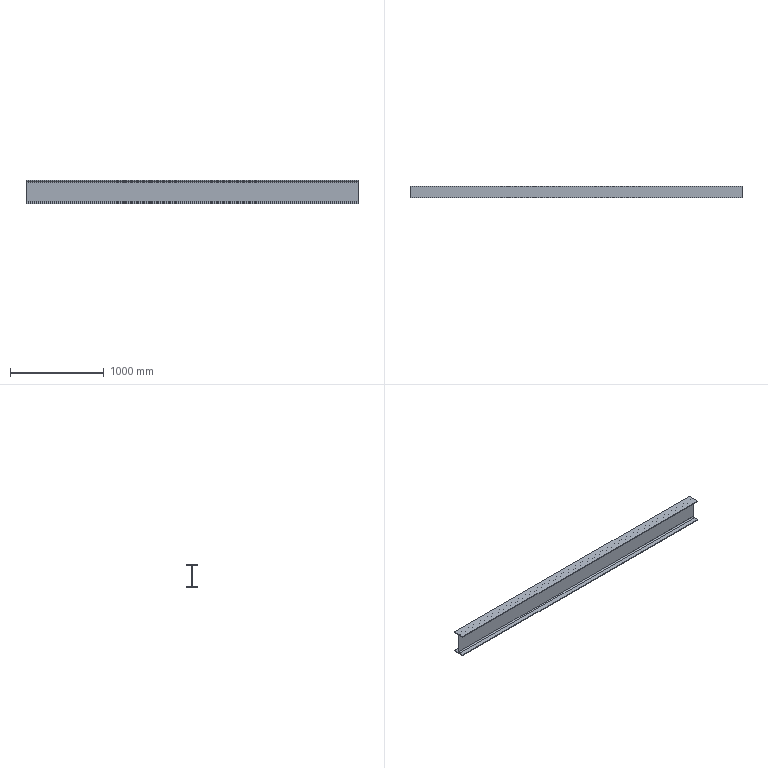Component | SolidWorks | H200X100-3600-13 | 1 solid | 18 faces | box 3550 x 125 x 250 mm | volume 12183851 mm3 | plane 14 | cylinder 4 | commonest cylinder face diameters 26 x4
build123d program:
from build123d import *

# Parameters (mm, degrees)
H_BEAM_HN200_100_1_DEPTH = 3550


with BuildPart() as part:
    # Sketch1 → H-beam HN200_100_1 (new body)
    with BuildSketch(Plane.YZ):
        with BuildLine():
            Line((-62.5, -125), (-62.5, -117))
            Line((-62.5, -117), (-15.75, -117))
            ThreePointArc((-15.75, -117), (-6.558, -113.192), (-2.75, -104))
            Line((-2.75, -104), (-2.75, 104))
            ThreePointArc((-2.75, 104), (-6.558, 113.192), (-15.75, 117))
            Line((-15.75, 117), (-62.5, 117))
            Line((-62.5, 117), (-62.5, 125))
            Line((-62.5, 125), (62.5, 125))
            Line((62.5, 125), (62.5, 117))
            Line((62.5, 117), (15.75, 117))
            ThreePointArc((15.75, 117), (6.558, 113.192), (2.75, 104))
            Line((2.75, 104), (2.75, -104))
            ThreePointArc((2.75, -104), (6.558, -113.192), (15.75, -117))
            Line((15.75, -117), (62.5, -117))
            Line((62.5, -117), (62.5, -125))
            Line((62.5, -125), (-62.5, -125))
        make_face()
    extrude(amount=H_BEAM_HN200_100_1_DEPTH)


solid = part.part

# Placed as in the assembly
solid = solid.moved(Location((-1730.074, -31202.346, 5154), (0, 0, 0)))
STEP:
#1=CARTESIAN_POINT('',(-68.113,-1230.899,197.992));
#2=VERTEX_POINT('',#1);
#3=CARTESIAN_POINT('',(-68.113,-1225.978,197.992));
#4=VERTEX_POINT('',#3);
#5=CARTESIAN_POINT('',(-68.113,-1225.978,197.992));
#6=DIRECTION('',(0.,1.,0.));
#7=VECTOR('',#6,39.37);
#8=LINE('',#5,#7);
#9=EDGE_CURVE('',#2,#4,#8,.T.);
#10=ORIENTED_EDGE('',*,*,#9,.T.);
#11=CARTESIAN_POINT('',(71.651,-1225.978,197.992));
#12=VERTEX_POINT('',#11);
#13=CARTESIAN_POINT('',(71.651,-1225.978,197.992));
#14=DIRECTION('',(-1.,0.,0.));
#15=VECTOR('',#14,39.37);
#16=LINE('',#13,#15);
#17=EDGE_CURVE('',#12,#4,#16,.T.);
#18=ORIENTED_EDGE('',*,*,#17,.F.);
#19=CARTESIAN_POINT('',(71.651,-1230.899,197.992));
#20=VERTEX_POINT('',#19);
#21=CARTESIAN_POINT('',(71.651,-1225.978,197.992));
#22=DIRECTION('',(0.,1.,0.));
#23=VECTOR('',#22,39.37);
#24=LINE('',#21,#23);
#25=EDGE_CURVE('',#20,#12,#24,.T.);
#26=ORIENTED_EDGE('',*,*,#25,.F.);
#27=CARTESIAN_POINT('',(71.651,-1230.899,197.992));
#28=DIRECTION('',(-1.,0.,0.));
#29=VECTOR('',#28,39.37);
#30=LINE('',#27,#29);
#31=EDGE_CURVE('',#20,#2,#30,.T.);
#32=ORIENTED_EDGE('',*,*,#31,.T.);
#33=EDGE_LOOP('',(#10,#18,#26,#32));
#34=FACE_OUTER_BOUND('',#33,.T.);
#35=CARTESIAN_POINT('',(71.651,-1225.978,197.992));
#36=DIRECTION('',(0.,0.,1.));
#37=DIRECTION('',(1.,0.,0.));
#38=AXIS2_PLACEMENT_3D('',#35,#36,#37);
#39=PLANE('',#38);
#40=ADVANCED_FACE('',(#34),#39,.F.);
#41=CARTESIAN_POINT('',(-68.113,-1225.978,198.307));
#42=VERTEX_POINT('',#41);
#43=CARTESIAN_POINT('',(-68.113,-1225.978,198.307));
#44=DIRECTION('',(0.,0.,1.));
#45=VECTOR('',#44,39.37);
#46=LINE('',#43,#45);
#47=EDGE_CURVE('',#4,#42,#46,.T.);
#48=ORIENTED_EDGE('',*,*,#47,.T.);
#49=CARTESIAN_POINT('',(71.651,-1225.978,198.307));
#50=VERTEX_POINT('',#49);
#51=CARTESIAN_POINT('',(71.651,-1225.978,198.307));
#52=DIRECTION('',(-1.,0.,0.));
#53=VECTOR('',#52,39.37);
#54=LINE('',#51,#53);
#55=EDGE_CURVE('',#50,#42,#54,.T.);
#56=ORIENTED_EDGE('',*,*,#55,.F.);
#57=CARTESIAN_POINT('',(71.651,-1225.978,198.307));
#58=DIRECTION('',(0.,0.,1.));
#59=VECTOR('',#58,39.37);
#60=LINE('',#57,#59);
#61=EDGE_CURVE('',#12,#50,#60,.T.);
#62=ORIENTED_EDGE('',*,*,#61,.F.);
#63=ORIENTED_EDGE('',*,*,#17,.T.);
#64=EDGE_LOOP('',(#48,#56,#62,#63));
#65=FACE_OUTER_BOUND('',#64,.T.);
#66=CARTESIAN_POINT('',(71.651,-1225.978,198.307));
#67=DIRECTION('',(0.,-1.,0.));
#68=DIRECTION('',(0.,0.,-1.));
#69=AXIS2_PLACEMENT_3D('',#66,#67,#68);
#70=PLANE('',#69);
#71=ADVANCED_FACE('',(#65),#70,.F.);
#72=CARTESIAN_POINT('',(-68.113,-1227.819,198.307));
#73=VERTEX_POINT('',#72);
#74=CARTESIAN_POINT('',(-68.113,-1225.978,198.307));
#75=DIRECTION('',(0.,-1.,0.));
#76=VECTOR('',#75,39.37);
#77=LINE('',#74,#76);
#78=EDGE_CURVE('',#42,#73,#77,.T.);
#79=ORIENTED_EDGE('',*,*,#78,.T.);
#80=CARTESIAN_POINT('',(71.651,-1227.819,198.307));
#81=VERTEX_POINT('',#80);
#82=CARTESIAN_POINT('',(71.651,-1227.819,198.307));
#83=DIRECTION('',(-1.,0.,0.));
#84=VECTOR('',#83,39.37);
#85=LINE('',#82,#84);
#86=EDGE_CURVE('',#81,#73,#85,.T.);
#87=ORIENTED_EDGE('',*,*,#86,.F.);
#88=CARTESIAN_POINT('',(71.651,-1225.978,198.307));
#89=DIRECTION('',(0.,-1.,0.));
#90=VECTOR('',#89,39.37);
#91=LINE('',#88,#90);
#92=EDGE_CURVE('',#50,#81,#91,.T.);
#93=ORIENTED_EDGE('',*,*,#92,.F.);
#94=ORIENTED_EDGE('',*,*,#55,.T.);
#95=EDGE_LOOP('',(#79,#87,#93,#94));
#96=FACE_OUTER_BOUND('',#95,.T.);
#97=CARTESIAN_POINT('',(71.651,-1225.978,198.307));
#98=DIRECTION('',(0.,0.,-1.));
#99=DIRECTION('',(-1.,0.,0.));
#100=AXIS2_PLACEMENT_3D('',#97,#98,#99);
#101=PLANE('',#100);
#102=ADVANCED_FACE('',(#96),#101,.F.);
#103=CARTESIAN_POINT('',(-68.113,-1228.331,198.819));
#104=VERTEX_POINT('',#103);
#105=CARTESIAN_POINT('',(-68.113,-1227.819,198.819));
#106=DIRECTION('',(-1.,0.,0.));
#107=DIRECTION('',(0.,0.,1.));
#108=AXIS2_PLACEMENT_3D('',#105,#106,#107);
#109=CIRCLE('',#108,0.5118);
#110=EDGE_CURVE('',#73,#104,#109,.T.);
#111=ORIENTED_EDGE('',*,*,#110,.T.);
#112=CARTESIAN_POINT('',(71.651,-1228.331,198.819));
#113=VERTEX_POINT('',#112);
#114=CARTESIAN_POINT('',(71.651,-1228.331,198.819));
#115=DIRECTION('',(-1.,0.,0.));
#116=VECTOR('',#115,39.37);
#117=LINE('',#114,#116);
#118=EDGE_CURVE('',#113,#104,#117,.T.);
#119=ORIENTED_EDGE('',*,*,#118,.F.);
#120=CARTESIAN_POINT('',(71.651,-1227.819,198.819));
#121=DIRECTION('',(-1.,0.,0.));
#122=DIRECTION('',(0.,0.,1.));
#123=AXIS2_PLACEMENT_3D('',#120,#121,#122);
#124=CIRCLE('',#123,0.5118);
#125=EDGE_CURVE('',#81,#113,#124,.T.);
#126=ORIENTED_EDGE('',*,*,#125,.F.);
#127=ORIENTED_EDGE('',*,*,#86,.T.);
#128=EDGE_LOOP('',(#111,#119,#126,#127));
#129=FACE_OUTER_BOUND('',#128,.T.);
#130=CARTESIAN_POINT('',(71.651,-1227.819,198.819));
#131=DIRECTION('',(-1.,0.,0.));
#132=DIRECTION('',(0.,0.,1.));
#133=AXIS2_PLACEMENT_3D('',#130,#131,#132);
#134=CYLINDRICAL_SURFACE('',#133,0.5118);
#135=ADVANCED_FACE('',(#129),#134,.F.);
#136=CARTESIAN_POINT('',(-68.113,-1228.331,207.008));
#137=VERTEX_POINT('',#136);
#138=CARTESIAN_POINT('',(-68.113,-1228.331,207.008));
#139=DIRECTION('',(0.,-0.,1.));
#140=VECTOR('',#139,39.37);
#141=LINE('',#138,#140);
#142=EDGE_CURVE('',#104,#137,#141,.T.);
#143=ORIENTED_EDGE('',*,*,#142,.T.);
#144=CARTESIAN_POINT('',(71.651,-1228.331,207.008));
#145=VERTEX_POINT('',#144);
#146=CARTESIAN_POINT('',(71.651,-1228.331,207.008));
#147=DIRECTION('',(-1.,0.,0.));
#148=VECTOR('',#147,39.37);
#149=LINE('',#146,#148);
#150=EDGE_CURVE('',#145,#137,#149,.T.);
#151=ORIENTED_EDGE('',*,*,#150,.F.);
#152=CARTESIAN_POINT('',(71.651,-1228.331,207.008));
#153=DIRECTION('',(0.,-0.,1.));
#154=VECTOR('',#153,39.37);
#155=LINE('',#152,#154);
#156=EDGE_CURVE('',#113,#145,#155,.T.);
#157=ORIENTED_EDGE('',*,*,#156,.F.);
#158=ORIENTED_EDGE('',*,*,#118,.T.);
#159=EDGE_LOOP('',(#143,#151,#157,#158));
#160=FACE_OUTER_BOUND('',#159,.T.);
#161=CARTESIAN_POINT('',(71.651,-1228.331,207.008));
#162=DIRECTION('',(0.,-1.,-0.));
#163=DIRECTION('',(0.,0.,-1.));
#164=AXIS2_PLACEMENT_3D('',#161,#162,#163);
#165=PLANE('',#164);
#166=ADVANCED_FACE('',(#160),#165,.F.);
#167=CARTESIAN_POINT('',(-68.113,-1227.819,207.52));
#168=VERTEX_POINT('',#167);
#169=CARTESIAN_POINT('',(-68.113,-1227.819,207.008));
#170=DIRECTION('',(-1.,0.,0.));
#171=DIRECTION('',(0.,0.,1.));
#172=AXIS2_PLACEMENT_3D('',#169,#170,#171);
#173=CIRCLE('',#172,0.5118);
#174=EDGE_CURVE('',#137,#168,#173,.T.);
#175=ORIENTED_EDGE('',*,*,#174,.T.);
#176=CARTESIAN_POINT('',(71.651,-1227.819,207.52));
#177=VERTEX_POINT('',#176);
#178=CARTESIAN_POINT('',(71.651,-1227.819,207.52));
#179=DIRECTION('',(-1.,0.,0.));
#180=VECTOR('',#179,39.37);
#181=LINE('',#178,#180);
#182=EDGE_CURVE('',#177,#168,#181,.T.);
#183=ORIENTED_EDGE('',*,*,#182,.F.);
#184=CARTESIAN_POINT('',(71.651,-1227.819,207.008));
#185=DIRECTION('',(-1.,0.,0.));
#186=DIRECTION('',(0.,0.,1.));
#187=AXIS2_PLACEMENT_3D('',#184,#185,#186);
#188=CIRCLE('',#187,0.5118);
#189=EDGE_CURVE('',#145,#177,#188,.T.);
#190=ORIENTED_EDGE('',*,*,#189,.F.);
#191=ORIENTED_EDGE('',*,*,#150,.T.);
#192=EDGE_LOOP('',(#175,#183,#190,#191));
#193=FACE_OUTER_BOUND('',#192,.T.);
#194=CARTESIAN_POINT('',(71.651,-1227.819,207.008));
#195=DIRECTION('',(-1.,0.,0.));
#196=DIRECTION('',(0.,0.,1.));
#197=AXIS2_PLACEMENT_3D('',#194,#195,#196);
#198=CYLINDRICAL_SURFACE('',#197,0.5118);
#199=ADVANCED_FACE('',(#193),#198,.F.);
#200=CARTESIAN_POINT('',(-68.113,-1225.978,207.52));
#201=VERTEX_POINT('',#200);
#202=CARTESIAN_POINT('',(-68.113,-1227.819,207.52));
#203=DIRECTION('',(0.,1.,0.));
#204=VECTOR('',#203,39.37);
#205=LINE('',#202,#204);
#206=EDGE_CURVE('',#168,#201,#205,.T.);
#207=ORIENTED_EDGE('',*,*,#206,.T.);
#208=CARTESIAN_POINT('',(71.651,-1225.978,207.52));
#209=VERTEX_POINT('',#208);
#210=CARTESIAN_POINT('',(71.651,-1225.978,207.52));
#211=DIRECTION('',(-1.,0.,0.));
#212=VECTOR('',#211,39.37);
#213=LINE('',#210,#212);
#214=EDGE_CURVE('',#209,#201,#213,.T.);
#215=ORIENTED_EDGE('',*,*,#214,.F.);
#216=CARTESIAN_POINT('',(71.651,-1227.819,207.52));
#217=DIRECTION('',(0.,1.,0.));
#218=VECTOR('',#217,39.37);
#219=LINE('',#216,#218);
#220=EDGE_CURVE('',#177,#209,#219,.T.);
#221=ORIENTED_EDGE('',*,*,#220,.F.);
#222=ORIENTED_EDGE('',*,*,#182,.T.);
#223=EDGE_LOOP('',(#207,#215,#221,#222));
#224=FACE_OUTER_BOUND('',#223,.T.);
#225=CARTESIAN_POINT('',(71.651,-1227.819,207.52));
#226=DIRECTION('',(0.,0.,1.));
#227=DIRECTION('',(1.,0.,0.));
#228=AXIS2_PLACEMENT_3D('',#225,#226,#227);
#229=PLANE('',#228);
#230=ADVANCED_FACE('',(#224),#229,.F.);
#231=CARTESIAN_POINT('',(-68.113,-1225.978,207.835));
#232=VERTEX_POINT('',#231);
#233=CARTESIAN_POINT('',(-68.113,-1225.978,207.835));
#234=DIRECTION('',(0.,0.,1.));
#235=VECTOR('',#234,39.37);
#236=LINE('',#233,#235);
#237=EDGE_CURVE('',#201,#232,#236,.T.);
#238=ORIENTED_EDGE('',*,*,#237,.T.);
#239=CARTESIAN_POINT('',(71.651,-1225.978,207.835));
#240=VERTEX_POINT('',#239);
#241=CARTESIAN_POINT('',(71.651,-1225.978,207.835));
#242=DIRECTION('',(-1.,0.,0.));
#243=VECTOR('',#242,39.37);
#244=LINE('',#241,#243);
#245=EDGE_CURVE('',#240,#232,#244,.T.);
#246=ORIENTED_EDGE('',*,*,#245,.F.);
#247=CARTESIAN_POINT('',(71.651,-1225.978,207.835));
#248=DIRECTION('',(0.,0.,1.));
#249=VECTOR('',#248,39.37);
#250=LINE('',#247,#249);
#251=EDGE_CURVE('',#209,#240,#250,.T.);
#252=ORIENTED_EDGE('',*,*,#251,.F.);
#253=ORIENTED_EDGE('',*,*,#214,.T.);
#254=EDGE_LOOP('',(#238,#246,#252,#253));
#255=FACE_OUTER_BOUND('',#254,.T.);
#256=CARTESIAN_POINT('',(71.651,-1225.978,207.835));
#257=DIRECTION('',(0.,-1.,0.));
#258=DIRECTION('',(0.,0.,-1.));
#259=AXIS2_PLACEMENT_3D('',#256,#257,#258);
#260=PLANE('',#259);
#261=ADVANCED_FACE('',(#255),#260,.F.);
#262=CARTESIAN_POINT('',(-68.113,-1230.899,207.835));
#263=VERTEX_POINT('',#262);
#264=CARTESIAN_POINT('',(-68.113,-1230.899,207.835));
#265=DIRECTION('',(0.,-1.,0.));
#266=VECTOR('',#265,39.37);
#267=LINE('',#264,#266);
#268=EDGE_CURVE('',#232,#263,#267,.T.);
#269=ORIENTED_EDGE('',*,*,#268,.T.);
#270=CARTESIAN_POINT('',(71.651,-1230.899,207.835));
#271=VERTEX_POINT('',#270);
#272=CARTESIAN_POINT('',(71.651,-1230.899,207.835));
#273=DIRECTION('',(-1.,0.,0.));
#274=VECTOR('',#273,39.37);
#275=LINE('',#272,#274);
#276=EDGE_CURVE('',#271,#263,#275,.T.);
#277=ORIENTED_EDGE('',*,*,#276,.F.);
#278=CARTESIAN_POINT('',(71.651,-1230.899,207.835));
#279=DIRECTION('',(0.,-1.,0.));
#280=VECTOR('',#279,39.37);
#281=LINE('',#278,#280);
#282=EDGE_CURVE('',#240,#271,#281,.T.);
#283=ORIENTED_EDGE('',*,*,#282,.F.);
#284=ORIENTED_EDGE('',*,*,#245,.T.);
#285=EDGE_LOOP('',(#269,#277,#283,#284));
#286=FACE_OUTER_BOUND('',#285,.T.);
#287=CARTESIAN_POINT('',(71.651,-1230.899,207.835));
#288=DIRECTION('',(0.,0.,-1.));
#289=DIRECTION('',(-1.,0.,0.));
#290=AXIS2_PLACEMENT_3D('',#287,#288,#289);
#291=PLANE('',#290);
#292=ADVANCED_FACE('',(#286),#291,.F.);
#293=CARTESIAN_POINT('',(-68.113,-1230.899,207.52));
#294=VERTEX_POINT('',#293);
#295=CARTESIAN_POINT('',(-68.113,-1230.899,207.52));
#296=DIRECTION('',(0.,0.,-1.));
#297=VECTOR('',#296,39.37);
#298=LINE('',#295,#297);
#299=EDGE_CURVE('',#263,#294,#298,.T.);
#300=ORIENTED_EDGE('',*,*,#299,.T.);
#301=CARTESIAN_POINT('',(71.651,-1230.899,207.52));
#302=VERTEX_POINT('',#301);
#303=CARTESIAN_POINT('',(71.651,-1230.899,207.52));
#304=DIRECTION('',(-1.,0.,0.));
#305=VECTOR('',#304,39.37);
#306=LINE('',#303,#305);
#307=EDGE_CURVE('',#302,#294,#306,.T.);
#308=ORIENTED_EDGE('',*,*,#307,.F.);
#309=CARTESIAN_POINT('',(71.651,-1230.899,207.52));
#310=DIRECTION('',(0.,0.,-1.));
#311=VECTOR('',#310,39.37);
#312=LINE('',#309,#311);
#313=EDGE_CURVE('',#271,#302,#312,.T.);
#314=ORIENTED_EDGE('',*,*,#313,.F.);
#315=ORIENTED_EDGE('',*,*,#276,.T.);
#316=EDGE_LOOP('',(#300,#308,#314,#315));
#317=FACE_OUTER_BOUND('',#316,.T.);
#318=CARTESIAN_POINT('',(71.651,-1230.899,207.52));
#319=DIRECTION('',(0.,1.,0.));
#320=DIRECTION('',(0.,0.,1.));
#321=AXIS2_PLACEMENT_3D('',#318,#319,#320);
#322=PLANE('',#321);
#323=ADVANCED_FACE('',(#317),#322,.F.);
#324=CARTESIAN_POINT('',(-68.113,-1229.059,207.52));
#325=VERTEX_POINT('',#324);
#326=CARTESIAN_POINT('',(-68.113,-1230.899,207.52));
#327=DIRECTION('',(0.,1.,0.));
#328=VECTOR('',#327,39.37);
#329=LINE('',#326,#328);
#330=EDGE_CURVE('',#294,#325,#329,.T.);
#331=ORIENTED_EDGE('',*,*,#330,.T.);
#332=CARTESIAN_POINT('',(71.651,-1229.059,207.52));
#333=VERTEX_POINT('',#332);
#334=CARTESIAN_POINT('',(71.651,-1229.059,207.52));
#335=DIRECTION('',(-1.,0.,0.));
#336=VECTOR('',#335,39.37);
#337=LINE('',#334,#336);
#338=EDGE_CURVE('',#333,#325,#337,.T.);
#339=ORIENTED_EDGE('',*,*,#338,.F.);
#340=CARTESIAN_POINT('',(71.651,-1230.899,207.52));
#341=DIRECTION('',(0.,1.,0.));
#342=VECTOR('',#341,39.37);
#343=LINE('',#340,#342);
#344=EDGE_CURVE('',#302,#333,#343,.T.);
#345=ORIENTED_EDGE('',*,*,#344,.F.);
#346=ORIENTED_EDGE('',*,*,#307,.T.);
#347=EDGE_LOOP('',(#331,#339,#345,#346));
#348=FACE_OUTER_BOUND('',#347,.T.);
#349=CARTESIAN_POINT('',(71.651,-1230.899,207.52));
#350=DIRECTION('',(0.,0.,1.));
#351=DIRECTION('',(1.,0.,0.));
#352=AXIS2_PLACEMENT_3D('',#349,#350,#351);
#353=PLANE('',#352);
#354=ADVANCED_FACE('',(#348),#353,.F.);
#355=CARTESIAN_POINT('',(-68.113,-1228.547,207.008));
#356=VERTEX_POINT('',#355);
#357=CARTESIAN_POINT('',(-68.113,-1229.059,207.008));
#358=DIRECTION('',(-1.,0.,0.));
#359=DIRECTION('',(0.,0.,-1.));
#360=AXIS2_PLACEMENT_3D('',#357,#358,#359);
#361=CIRCLE('',#360,0.5118);
#362=EDGE_CURVE('',#325,#356,#361,.T.);
#363=ORIENTED_EDGE('',*,*,#362,.T.);
#364=CARTESIAN_POINT('',(71.651,-1228.547,207.008));
#365=VERTEX_POINT('',#364);
#366=CARTESIAN_POINT('',(71.651,-1228.547,207.008));
#367=DIRECTION('',(-1.,0.,0.));
#368=VECTOR('',#367,39.37);
#369=LINE('',#366,#368);
#370=EDGE_CURVE('',#365,#356,#369,.T.);
#371=ORIENTED_EDGE('',*,*,#370,.F.);
#372=CARTESIAN_POINT('',(71.651,-1229.059,207.008));
#373=DIRECTION('',(-1.,0.,0.));
#374=DIRECTION('',(0.,0.,-1.));
#375=AXIS2_PLACEMENT_3D('',#372,#373,#374);
#376=CIRCLE('',#375,0.5118);
#377=EDGE_CURVE('',#333,#365,#376,.T.);
#378=ORIENTED_EDGE('',*,*,#377,.F.);
#379=ORIENTED_EDGE('',*,*,#338,.T.);
#380=EDGE_LOOP('',(#363,#371,#378,#379));
#381=FACE_OUTER_BOUND('',#380,.T.);
#382=CARTESIAN_POINT('',(71.651,-1229.059,207.008));
#383=DIRECTION('',(-1.,0.,0.));
#384=DIRECTION('',(0.,0.,1.));
#385=AXIS2_PLACEMENT_3D('',#382,#383,#384);
#386=CYLINDRICAL_SURFACE('',#385,0.5118);
#387=ADVANCED_FACE('',(#381),#386,.F.);
#388=CARTESIAN_POINT('',(-68.113,-1228.547,198.819));
#389=VERTEX_POINT('',#388);
#390=CARTESIAN_POINT('',(-68.113,-1228.547,198.819));
#391=DIRECTION('',(0.,0.,-1.));
#392=VECTOR('',#391,39.37);
#393=LINE('',#390,#392);
#394=EDGE_CURVE('',#356,#389,#393,.T.);
#395=ORIENTED_EDGE('',*,*,#394,.T.);
#396=CARTESIAN_POINT('',(71.651,-1228.547,198.819));
#397=VERTEX_POINT('',#396);
#398=CARTESIAN_POINT('',(71.651,-1228.547,198.819));
#399=DIRECTION('',(-1.,0.,0.));
#400=VECTOR('',#399,39.37);
#401=LINE('',#398,#400);
#402=EDGE_CURVE('',#397,#389,#401,.T.);
#403=ORIENTED_EDGE('',*,*,#402,.F.);
#404=CARTESIAN_POINT('',(71.651,-1228.547,198.819));
#405=DIRECTION('',(0.,0.,-1.));
#406=VECTOR('',#405,39.37);
#407=LINE('',#404,#406);
#408=EDGE_CURVE('',#365,#397,#407,.T.);
#409=ORIENTED_EDGE('',*,*,#408,.F.);
#410=ORIENTED_EDGE('',*,*,#370,.T.);
#411=EDGE_LOOP('',(#395,#403,#409,#410));
#412=FACE_OUTER_BOUND('',#411,.T.);
#413=CARTESIAN_POINT('',(71.651,-1228.547,198.819));
#414=DIRECTION('',(0.,1.,0.));
#415=DIRECTION('',(0.,-0.,1.));
#416=AXIS2_PLACEMENT_3D('',#413,#414,#415);
#417=PLANE('',#416);
#418=ADVANCED_FACE('',(#412),#417,.F.);
#419=CARTESIAN_POINT('',(-68.113,-1229.059,198.307));
#420=VERTEX_POINT('',#419);
#421=CARTESIAN_POINT('',(-68.113,-1229.059,198.819));
#422=DIRECTION('',(-1.,0.,0.));
#423=DIRECTION('',(0.,0.,-1.));
#424=AXIS2_PLACEMENT_3D('',#421,#422,#423);
#425=CIRCLE('',#424,0.5118);
#426=EDGE_CURVE('',#389,#420,#425,.T.);
#427=ORIENTED_EDGE('',*,*,#426,.T.);
#428=CARTESIAN_POINT('',(71.651,-1229.059,198.307));
#429=VERTEX_POINT('',#428);
#430=CARTESIAN_POINT('',(71.651,-1229.059,198.307));
#431=DIRECTION('',(-1.,0.,0.));
#432=VECTOR('',#431,39.37);
#433=LINE('',#430,#432);
#434=EDGE_CURVE('',#429,#420,#433,.T.);
#435=ORIENTED_EDGE('',*,*,#434,.F.);
#436=CARTESIAN_POINT('',(71.651,-1229.059,198.819));
#437=DIRECTION('',(-1.,0.,0.));
#438=DIRECTION('',(0.,0.,-1.));
#439=AXIS2_PLACEMENT_3D('',#436,#437,#438);
#440=CIRCLE('',#439,0.5118);
#441=EDGE_CURVE('',#397,#429,#440,.T.);
#442=ORIENTED_EDGE('',*,*,#441,.F.);
#443=ORIENTED_EDGE('',*,*,#402,.T.);
#444=EDGE_LOOP('',(#427,#435,#442,#443));
#445=FACE_OUTER_BOUND('',#444,.T.);
#446=CARTESIAN_POINT('',(71.651,-1229.059,198.819));
#447=DIRECTION('',(-1.,0.,0.));
#448=DIRECTION('',(0.,0.,1.));
#449=AXIS2_PLACEMENT_3D('',#446,#447,#448);
#450=CYLINDRICAL_SURFACE('',#449,0.5118);
#451=ADVANCED_FACE('',(#445),#450,.F.);
#452=CARTESIAN_POINT('',(-68.113,-1230.899,198.307));
#453=VERTEX_POINT('',#452);
#454=CARTESIAN_POINT('',(-68.113,-1229.059,198.307));
#455=DIRECTION('',(0.,-1.,0.));
#456=VECTOR('',#455,39.37);
#457=LINE('',#454,#456);
#458=EDGE_CURVE('',#420,#453,#457,.T.);
#459=ORIENTED_EDGE('',*,*,#458,.T.);
#460=CARTESIAN_POINT('',(71.651,-1230.899,198.307));
#461=VERTEX_POINT('',#460);
#462=CARTESIAN_POINT('',(71.651,-1230.899,198.307));
#463=DIRECTION('',(-1.,0.,0.));
#464=VECTOR('',#463,39.37);
#465=LINE('',#462,#464);
#466=EDGE_CURVE('',#461,#453,#465,.T.);
#467=ORIENTED_EDGE('',*,*,#466,.F.);
#468=CARTESIAN_POINT('',(71.651,-1229.059,198.307));
#469=DIRECTION('',(0.,-1.,0.));
#470=VECTOR('',#469,39.37);
#471=LINE('',#468,#470);
#472=EDGE_CURVE('',#429,#461,#471,.T.);
#473=ORIENTED_EDGE('',*,*,#472,.F.);
#474=ORIENTED_EDGE('',*,*,#434,.T.);
#475=EDGE_LOOP('',(#459,#467,#473,#474));
#476=FACE_OUTER_BOUND('',#475,.T.);
#477=CARTESIAN_POINT('',(71.651,-1229.059,198.307));
#478=DIRECTION('',(0.,0.,-1.));
#479=DIRECTION('',(-1.,0.,0.));
#480=AXIS2_PLACEMENT_3D('',#477,#478,#479);
#481=PLANE('',#480);
#482=ADVANCED_FACE('',(#476),#481,.F.);
#483=CARTESIAN_POINT('',(-68.113,-1230.899,197.992));
#484=DIRECTION('',(0.,0.,-1.));
#485=VECTOR('',#484,39.37);
#486=LINE('',#483,#485);
#487=EDGE_CURVE('',#453,#2,#486,.T.);
#488=ORIENTED_EDGE('',*,*,#487,.T.);
#489=ORIENTED_EDGE('',*,*,#31,.F.);
#490=CARTESIAN_POINT('',(71.651,-1230.899,197.992));
#491=DIRECTION('',(0.,0.,-1.));
#492=VECTOR('',#491,39.37);
#493=LINE('',#490,#492);
#494=EDGE_CURVE('',#461,#20,#493,.T.);
#495=ORIENTED_EDGE('',*,*,#494,.F.);
#496=ORIENTED_EDGE('',*,*,#466,.T.);
#497=EDGE_LOOP('',(#488,#489,#495,#496));
#498=FACE_OUTER_BOUND('',#497,.T.);
#499=CARTESIAN_POINT('',(71.651,-1230.899,197.992));
#500=DIRECTION('',(0.,1.,0.));
#501=DIRECTION('',(0.,0.,1.));
#502=AXIS2_PLACEMENT_3D('',#499,#500,#501);
#503=PLANE('',#502);
#504=ADVANCED_FACE('',(#498),#503,.F.);
#505=ORIENTED_EDGE('',*,*,#25,.T.);
#506=ORIENTED_EDGE('',*,*,#61,.T.);
#507=ORIENTED_EDGE('',*,*,#92,.T.);
#508=ORIENTED_EDGE('',*,*,#125,.T.);
#509=ORIENTED_EDGE('',*,*,#156,.T.);
#510=ORIENTED_EDGE('',*,*,#189,.T.);
#511=ORIENTED_EDGE('',*,*,#220,.T.);
#512=ORIENTED_EDGE('',*,*,#251,.T.);
#513=ORIENTED_EDGE('',*,*,#282,.T.);
#514=ORIENTED_EDGE('',*,*,#313,.T.);
#515=ORIENTED_EDGE('',*,*,#344,.T.);
#516=ORIENTED_EDGE('',*,*,#377,.T.);
#517=ORIENTED_EDGE('',*,*,#408,.T.);
#518=ORIENTED_EDGE('',*,*,#441,.T.);
#519=ORIENTED_EDGE('',*,*,#472,.T.);
#520=ORIENTED_EDGE('',*,*,#494,.T.);
#521=EDGE_LOOP('',(#505,#506,#507,#508,#509,#510,#511,#512,#513,#514,#515,#516,#517,#518,#519,#520));
#522=FACE_OUTER_BOUND('',#521,.T.);
#523=CARTESIAN_POINT('',(71.651,-1229.059,198.819));
#524=DIRECTION('',(1.,0.,0.));
#525=DIRECTION('',(0.,0.,-1.));
#526=AXIS2_PLACEMENT_3D('',#523,#524,#525);
#527=PLANE('',#526);
#528=ADVANCED_FACE('',(#522),#527,.T.);
#529=ORIENTED_EDGE('',*,*,#9,.F.);
#530=ORIENTED_EDGE('',*,*,#487,.F.);
#531=ORIENTED_EDGE('',*,*,#458,.F.);
#532=ORIENTED_EDGE('',*,*,#426,.F.);
#533=ORIENTED_EDGE('',*,*,#394,.F.);
#534=ORIENTED_EDGE('',*,*,#362,.F.);
#535=ORIENTED_EDGE('',*,*,#330,.F.);
#536=ORIENTED_EDGE('',*,*,#299,.F.);
#537=ORIENTED_EDGE('',*,*,#268,.F.);
#538=ORIENTED_EDGE('',*,*,#237,.F.);
#539=ORIENTED_EDGE('',*,*,#206,.F.);
#540=ORIENTED_EDGE('',*,*,#174,.F.);
#541=ORIENTED_EDGE('',*,*,#142,.F.);
#542=ORIENTED_EDGE('',*,*,#110,.F.);
#543=ORIENTED_EDGE('',*,*,#78,.F.);
#544=ORIENTED_EDGE('',*,*,#47,.F.);
#545=EDGE_LOOP('',(#529,#530,#531,#532,#533,#534,#535,#536,#537,#538,#539,#540,#541,#542,#543,#544));
#546=FACE_OUTER_BOUND('',#545,.T.);
#547=CARTESIAN_POINT('',(-68.113,-1229.059,198.819));
#548=DIRECTION('',(1.,0.,0.));
#549=DIRECTION('',(0.,0.,-1.));
#550=AXIS2_PLACEMENT_3D('',#547,#548,#549);
#551=PLANE('',#550);
#552=ADVANCED_FACE('',(#546),#551,.F.);
#553=CLOSED_SHELL('',(#40,#71,#102,#135,#166,#199,#230,#261,#292,#323,#354,#387,#418,#451,#482,#504,#528,#552));
#554=MANIFOLD_SOLID_BREP('',#553);
#555=CARTESIAN_POINT('',(0.,0.,0.));
#556=DIRECTION('',(0.,0.,1.));
#557=DIRECTION('',(1.,0.,0.));
#558=AXIS2_PLACEMENT_3D('',#555,#556,#557);
#559=(LENGTH_UNIT()NAMED_UNIT(*)SI_UNIT($,.METRE.));
#560=LENGTH_MEASURE_WITH_UNIT(LENGTH_MEASURE(0.0254),#559);
#561=DIMENSIONAL_EXPONENTS(1.,0.,0.,0.,0.,0.,0.);
#562=(CONVERSION_BASED_UNIT('',#560)LENGTH_UNIT()NAMED_UNIT(#561));
#563=UNCERTAINTY_MEASURE_WITH_UNIT(LENGTH_MEASURE(0.00001),#562,'','');
#564=(NAMED_UNIT(*)PLANE_ANGLE_UNIT()SI_UNIT($,.RADIAN.));
#565=(NAMED_UNIT(*)SI_UNIT($,.STERADIAN.)SOLID_ANGLE_UNIT());
#566=(GEOMETRIC_REPRESENTATION_CONTEXT(3)GLOBAL_UNCERTAINTY_ASSIGNED_CONTEXT((#563))GLOBAL_UNIT_ASSIGNED_CONTEXT((#562,#564,#565))REPRESENTATION_CONTEXT('',''));
#567=ADVANCED_BREP_SHAPE_REPRESENTATION('',(#554,#558),#566);
#568=COLOUR_RGB('',0.7922,0.8196,0.9333);
#569=FILL_AREA_STYLE_COLOUR('',#568);
#570=FILL_AREA_STYLE('',(#569));
#571=SURFACE_STYLE_FILL_AREA(#570);
#572=SURFACE_SIDE_STYLE('',(#571));
#573=SURFACE_STYLE_USAGE(.BOTH.,#572);
#574=PRESENTATION_STYLE_ASSIGNMENT((#573));
#575=STYLED_ITEM('',(#574),#554);
#576=PRESENTATION_LAYER_ASSIGNMENT('','',(#575));
#577=(LENGTH_UNIT()NAMED_UNIT(*)SI_UNIT($,.METRE.));
#578=LENGTH_MEASURE_WITH_UNIT(LENGTH_MEASURE(0.0254),#577);
#579=DIMENSIONAL_EXPONENTS(1.,0.,0.,0.,0.,0.,0.);
#580=(CONVERSION_BASED_UNIT('',#578)LENGTH_UNIT()NAMED_UNIT(#579));
#581=UNCERTAINTY_MEASURE_WITH_UNIT(LENGTH_MEASURE(0.00001),#580,'','');
#582=(NAMED_UNIT(*)PLANE_ANGLE_UNIT()SI_UNIT($,.RADIAN.));
#583=(NAMED_UNIT(*)SI_UNIT($,.STERADIAN.)SOLID_ANGLE_UNIT());
#584=(GEOMETRIC_REPRESENTATION_CONTEXT(3)GLOBAL_UNCERTAINTY_ASSIGNED_CONTEXT((#581))GLOBAL_UNIT_ASSIGNED_CONTEXT((#580,#582,#583))REPRESENTATION_CONTEXT('',''));
#585=MECHANICAL_DESIGN_GEOMETRIC_PRESENTATION_REPRESENTATION('',(#575),#584);